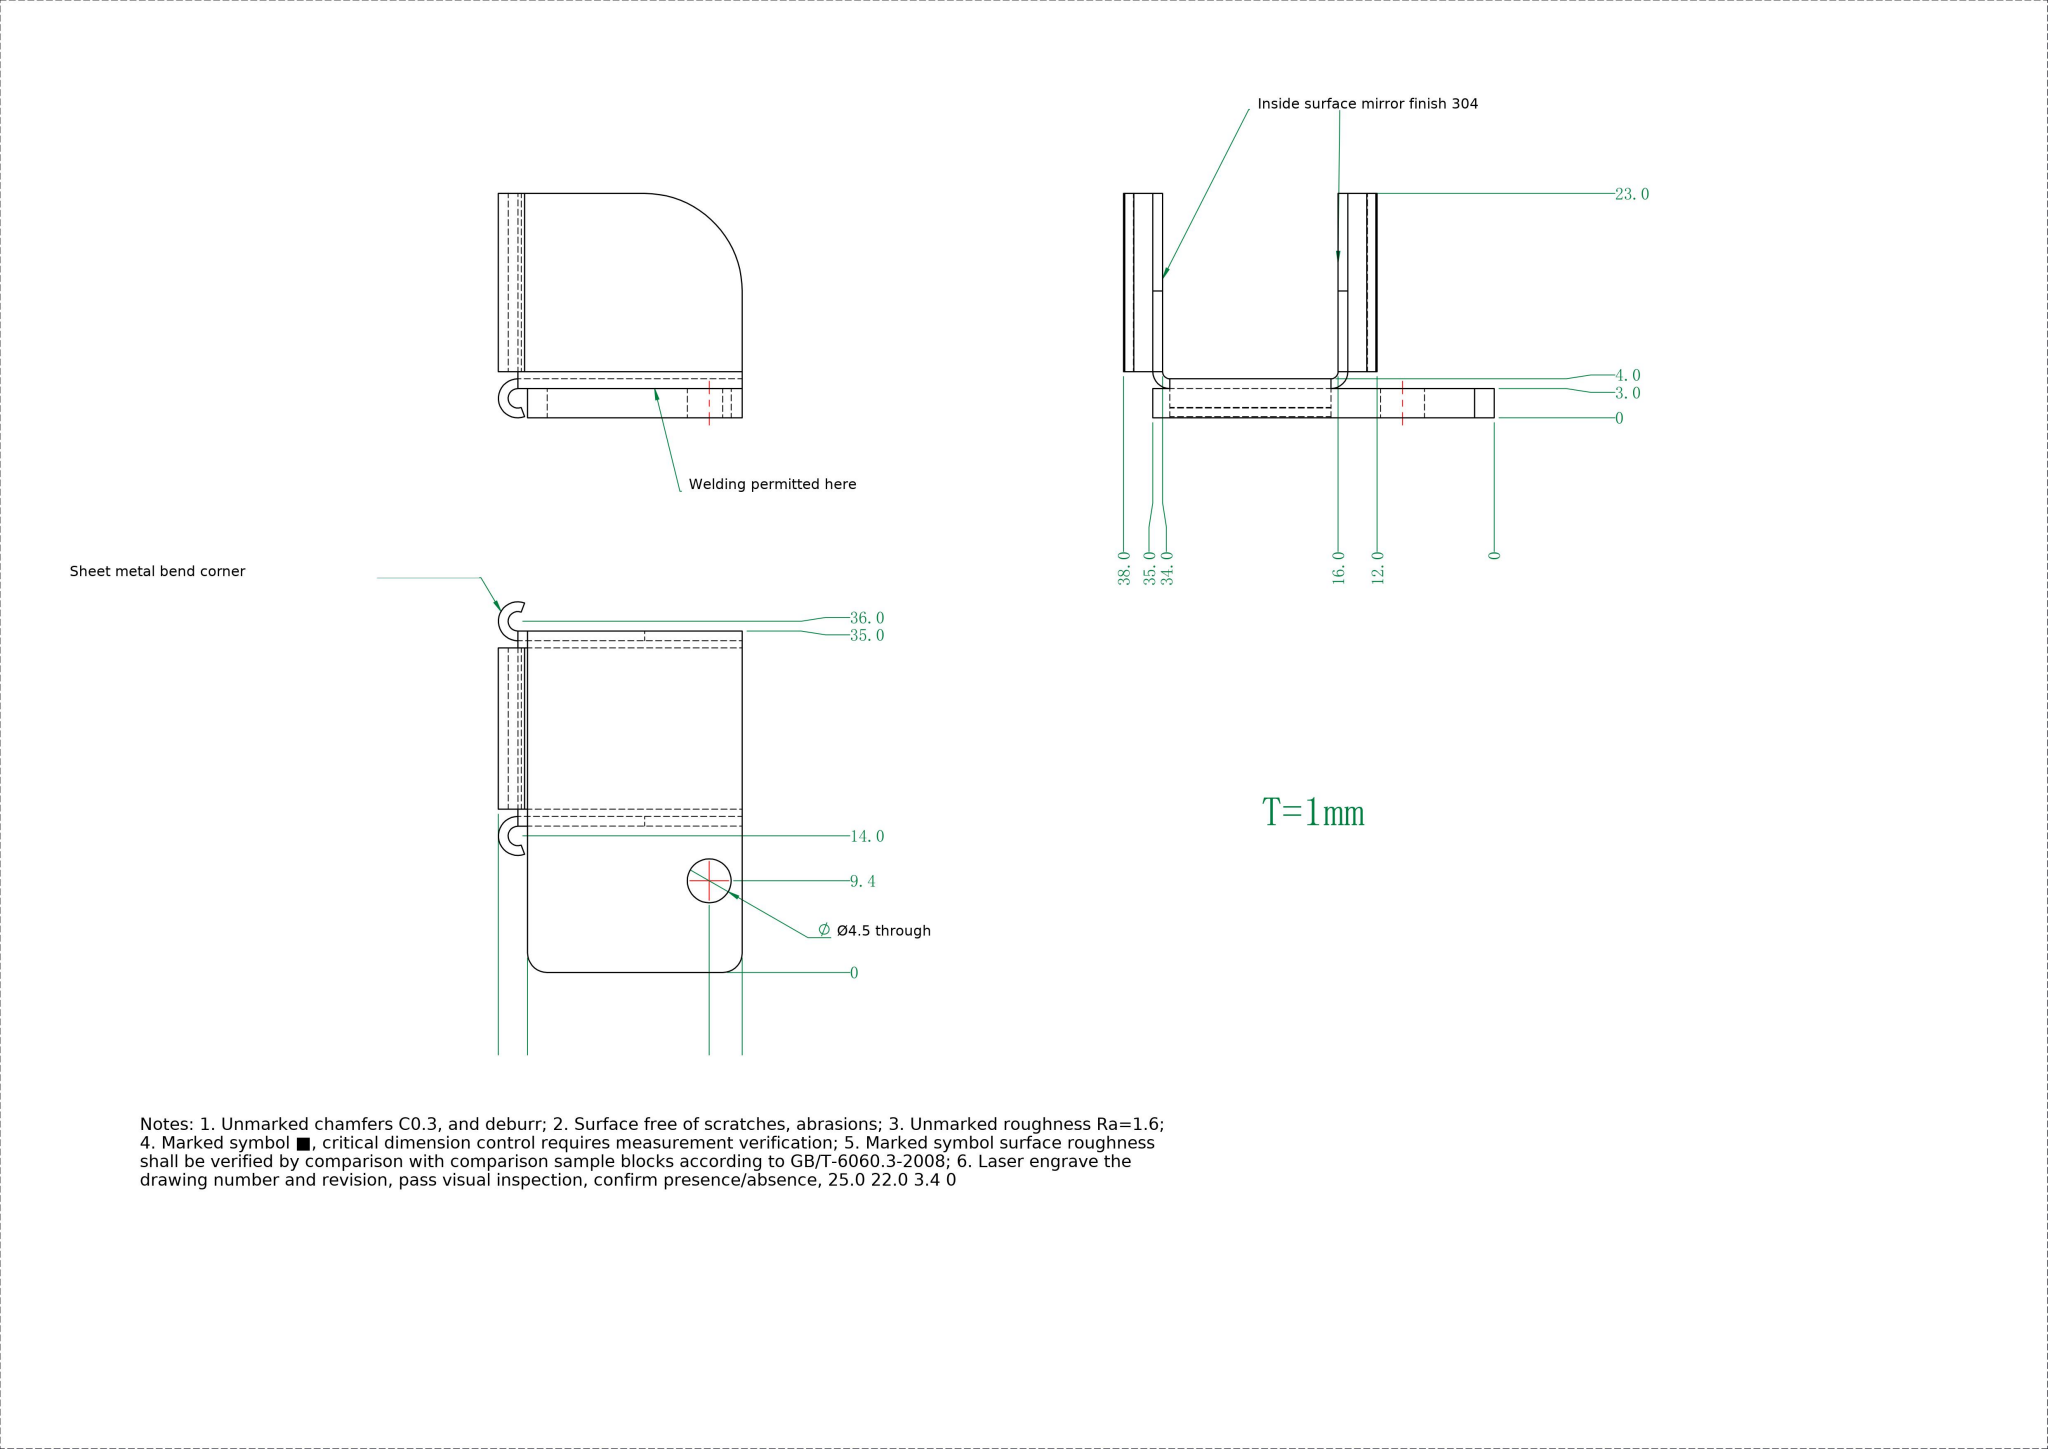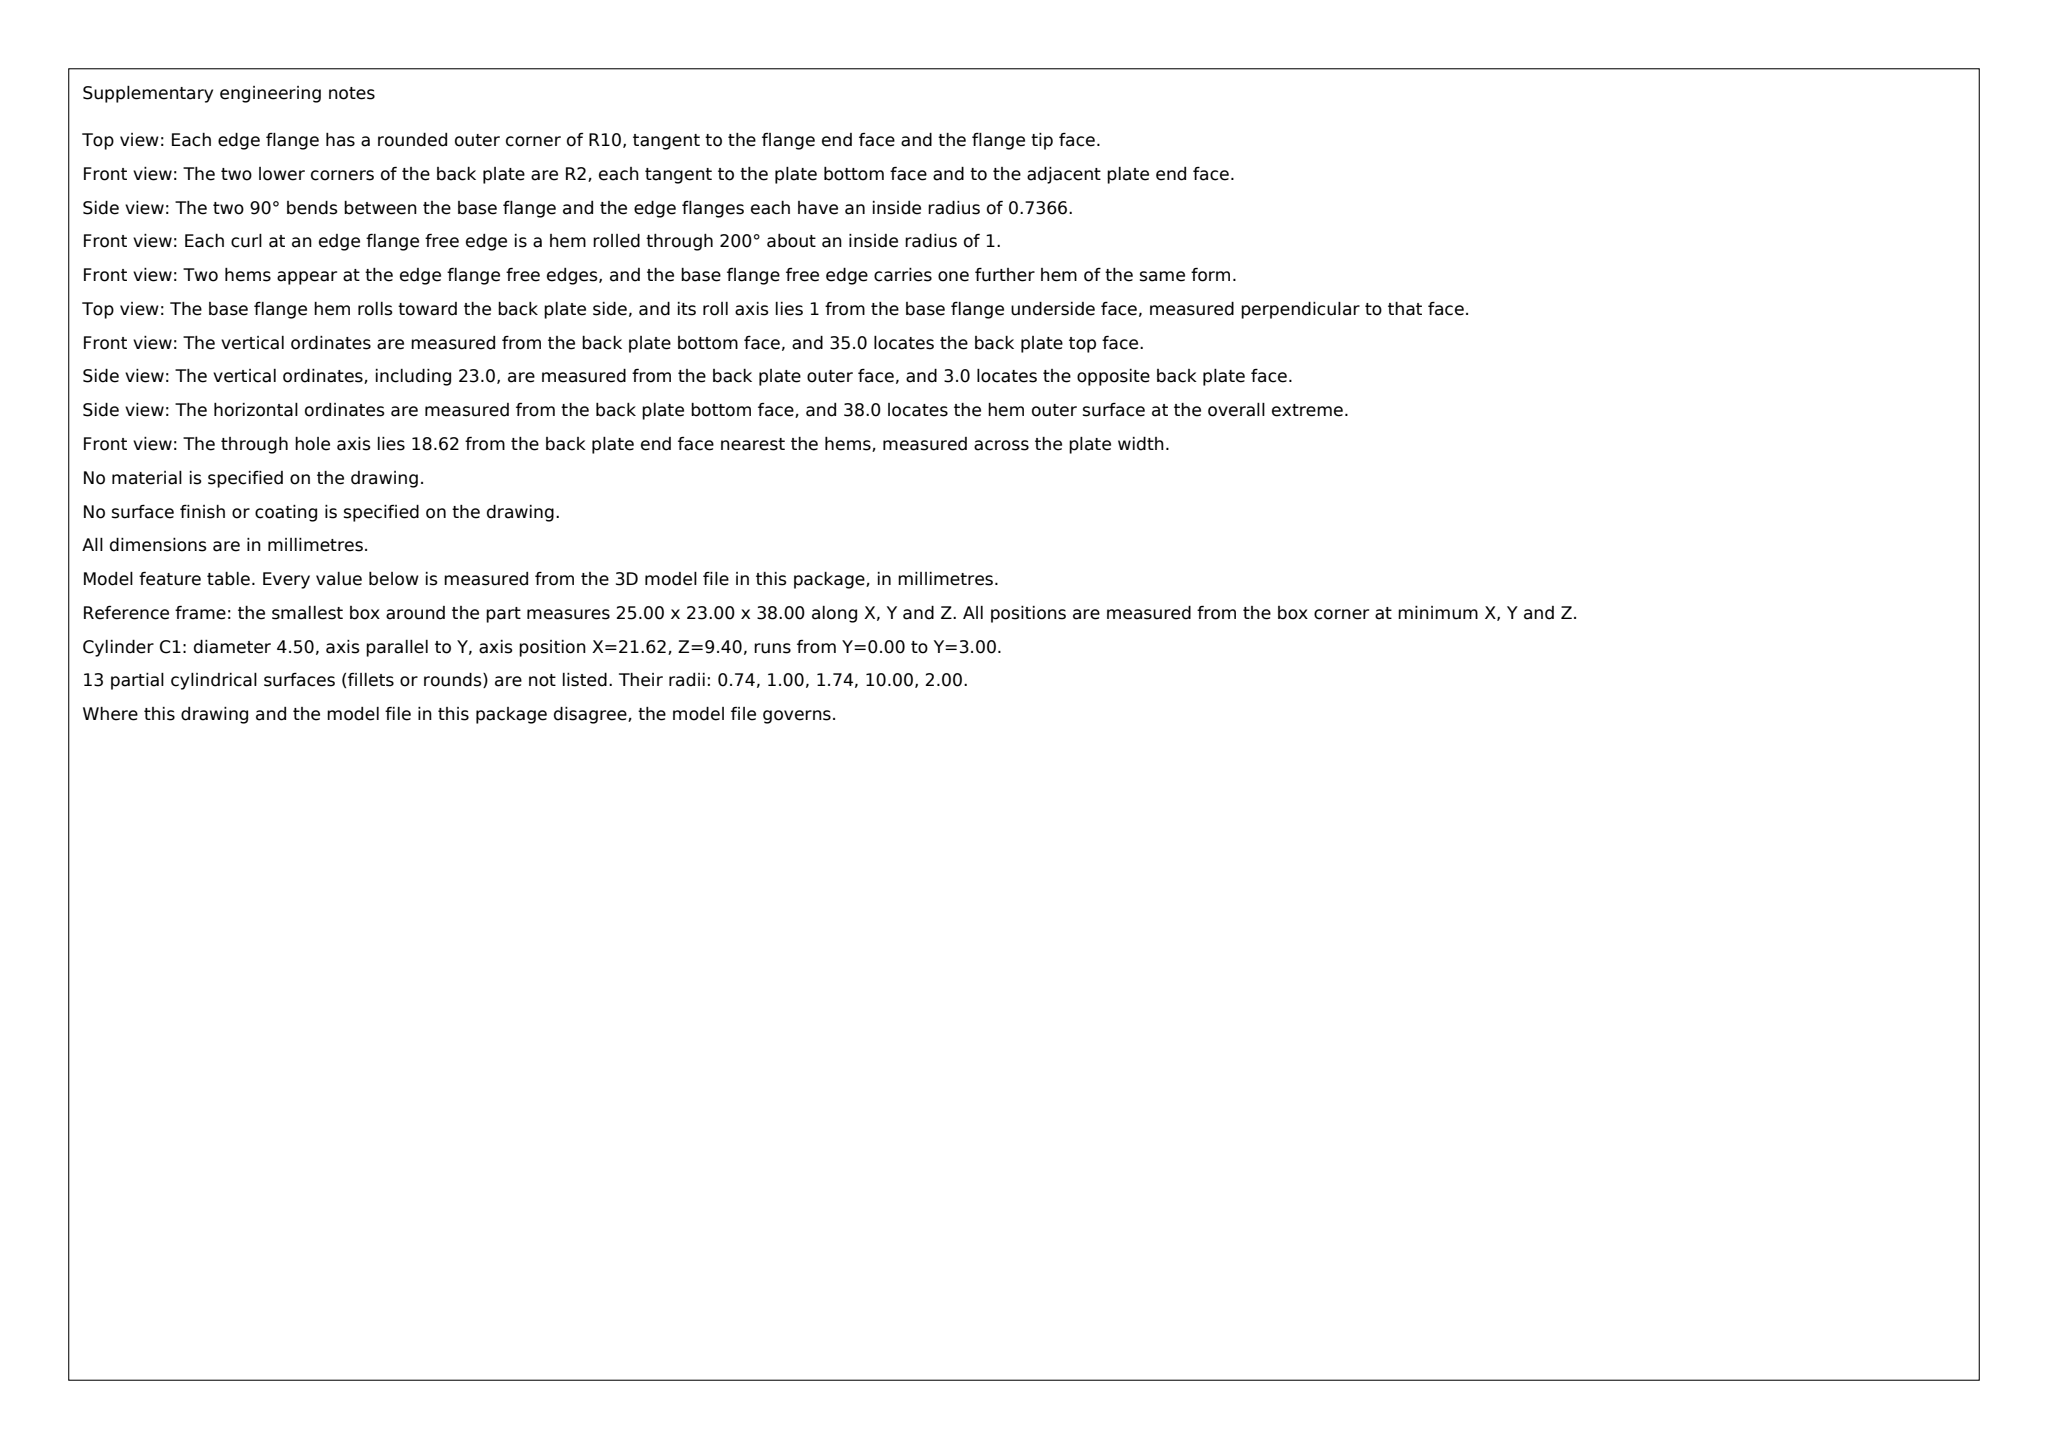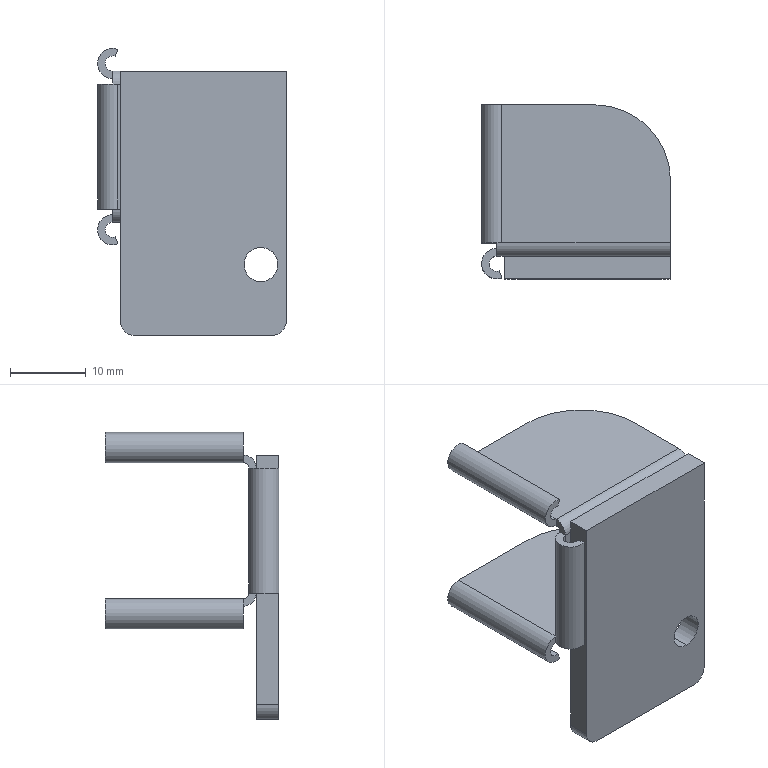Part | SolidWorks | mm | material 304 | 1 solid | 46 faces | box 25 x 23 x 38 mm | volume 3802 mm3 | plane 30 | cylinder 16 | commonest cylinder face diameters 4 x5 2 x3 4.5 x2 3.473 x2 1.473 x2 20 x2
Drawing notes:
OVERALL WIDTH 25.0 IN X (TOP & FRONT VIEWS) | from the solid: bbox_xyz X = 25.0; planes x=0 and x=25.0
HEMMED BEND CORNERS AT Z14 & Z36: R1 INR / R2 OTR | from the solid: cyl dia 2.0 & dia 4.0 axis y at x=2.0, z=14.0 and z=36.0
R2 VERT CORNER AT X2,Y2, 16.6 HIGH | from the solid: convex arc (round/outer radius) dia 4.0, axis z, axis_pos [2.0, 2.0], from z=16.7 to z=33.3 (with matching concave dia 2.0 arc) -> corner height = 33.3-16.7 = 16.6
1X Ø4.5 THRU ONLY AT 21.6 FROM LH EDGE, 9.4 FROM 0 - DEL 2X | from the solid: hole/bore dia 4.5 axis y at [21.6, z9.4] from 0.0 to 3.0, count 1 (no second hole)
HEM/SHELF FACE 4.7 FROM 0 FACE (0.7 BEYOND 4. 0 FACE) | from the solid: planes y=0.0, y=3.0, y=4.0 and y=4.7 (x0-2.7, z12-16 / z34-38); arcs start y=4.7
HEM RETURNS: 20° FACES, 0.9 OFFSET, AT Z16.7 & Z33.3, Y4.7 | from the solid: inclined planes 20°: from [2.3,0.1,16.7] sz [0.3,0.9,16.5]; [2.3,4.7,12.1] & [2.3,4.7,36.9] sz [0.3,18.3,0.9]
VERT R2 CORNER/INNER WEB: Z16.7 TO Z33.3 = 16.6 HIGH | from the solid: arcs dia 2.0/4.0 axis z at [2.0,2.0] from 16.7 to 33.3; plane y=3.0 x2-3 z16.7-33.3; plane y=4.0 z16.7-33.3
NOTE 6: DEL STRAY 22. 0/3. 4/0; OVERALL 25. 0 x 23. 0 x 38. 0 | from the solid: bbox_xyz [25.0, 23.0, 38.0]